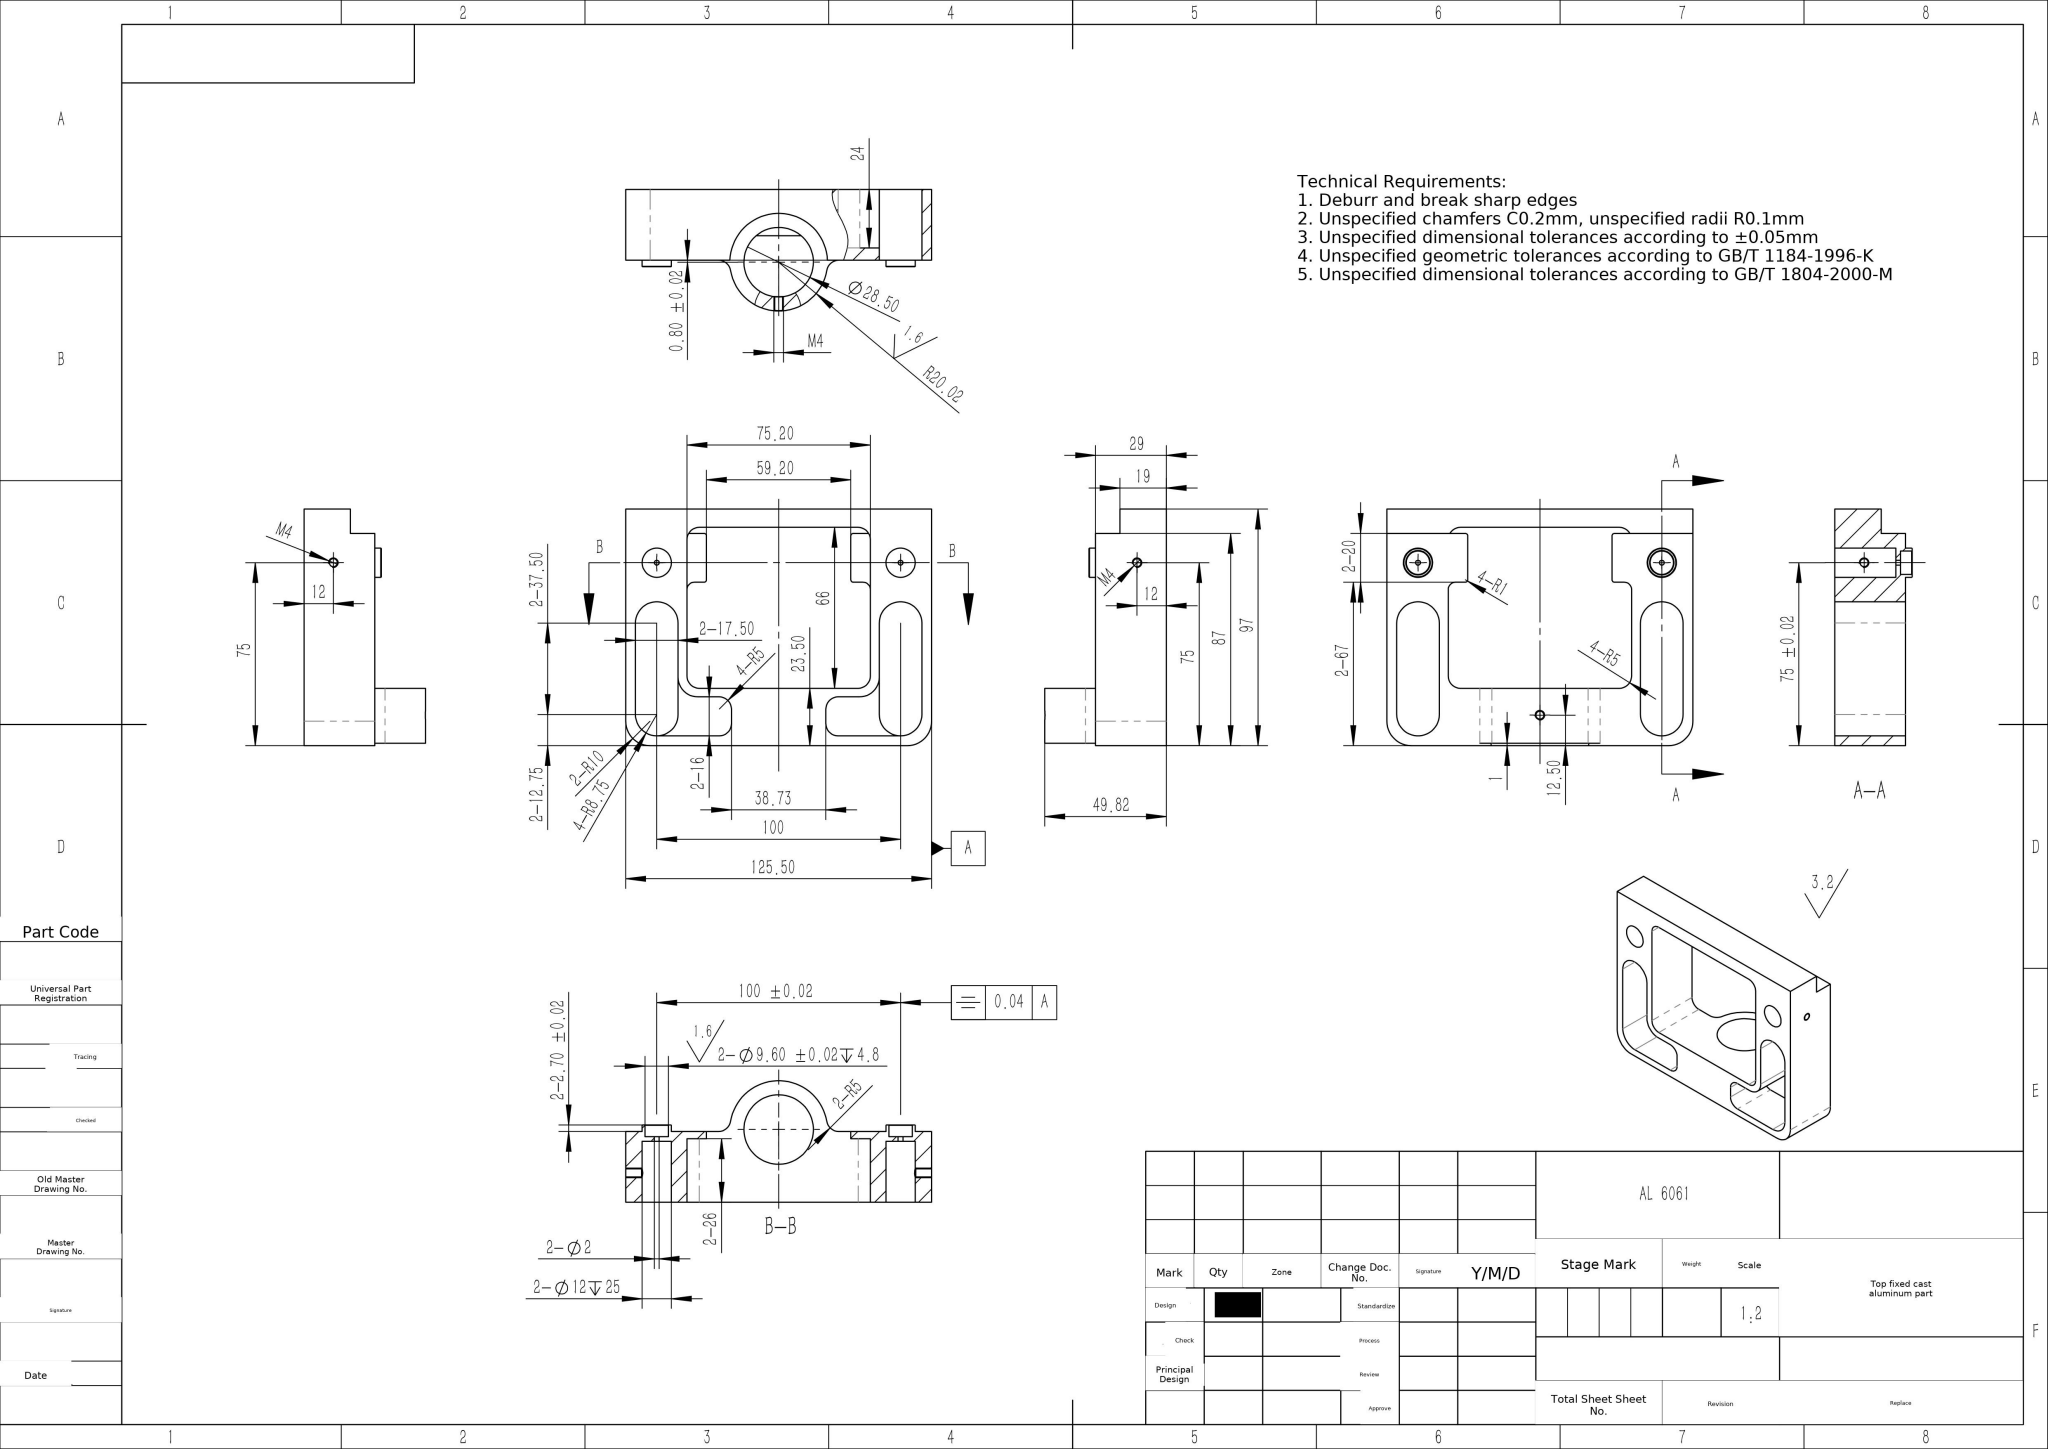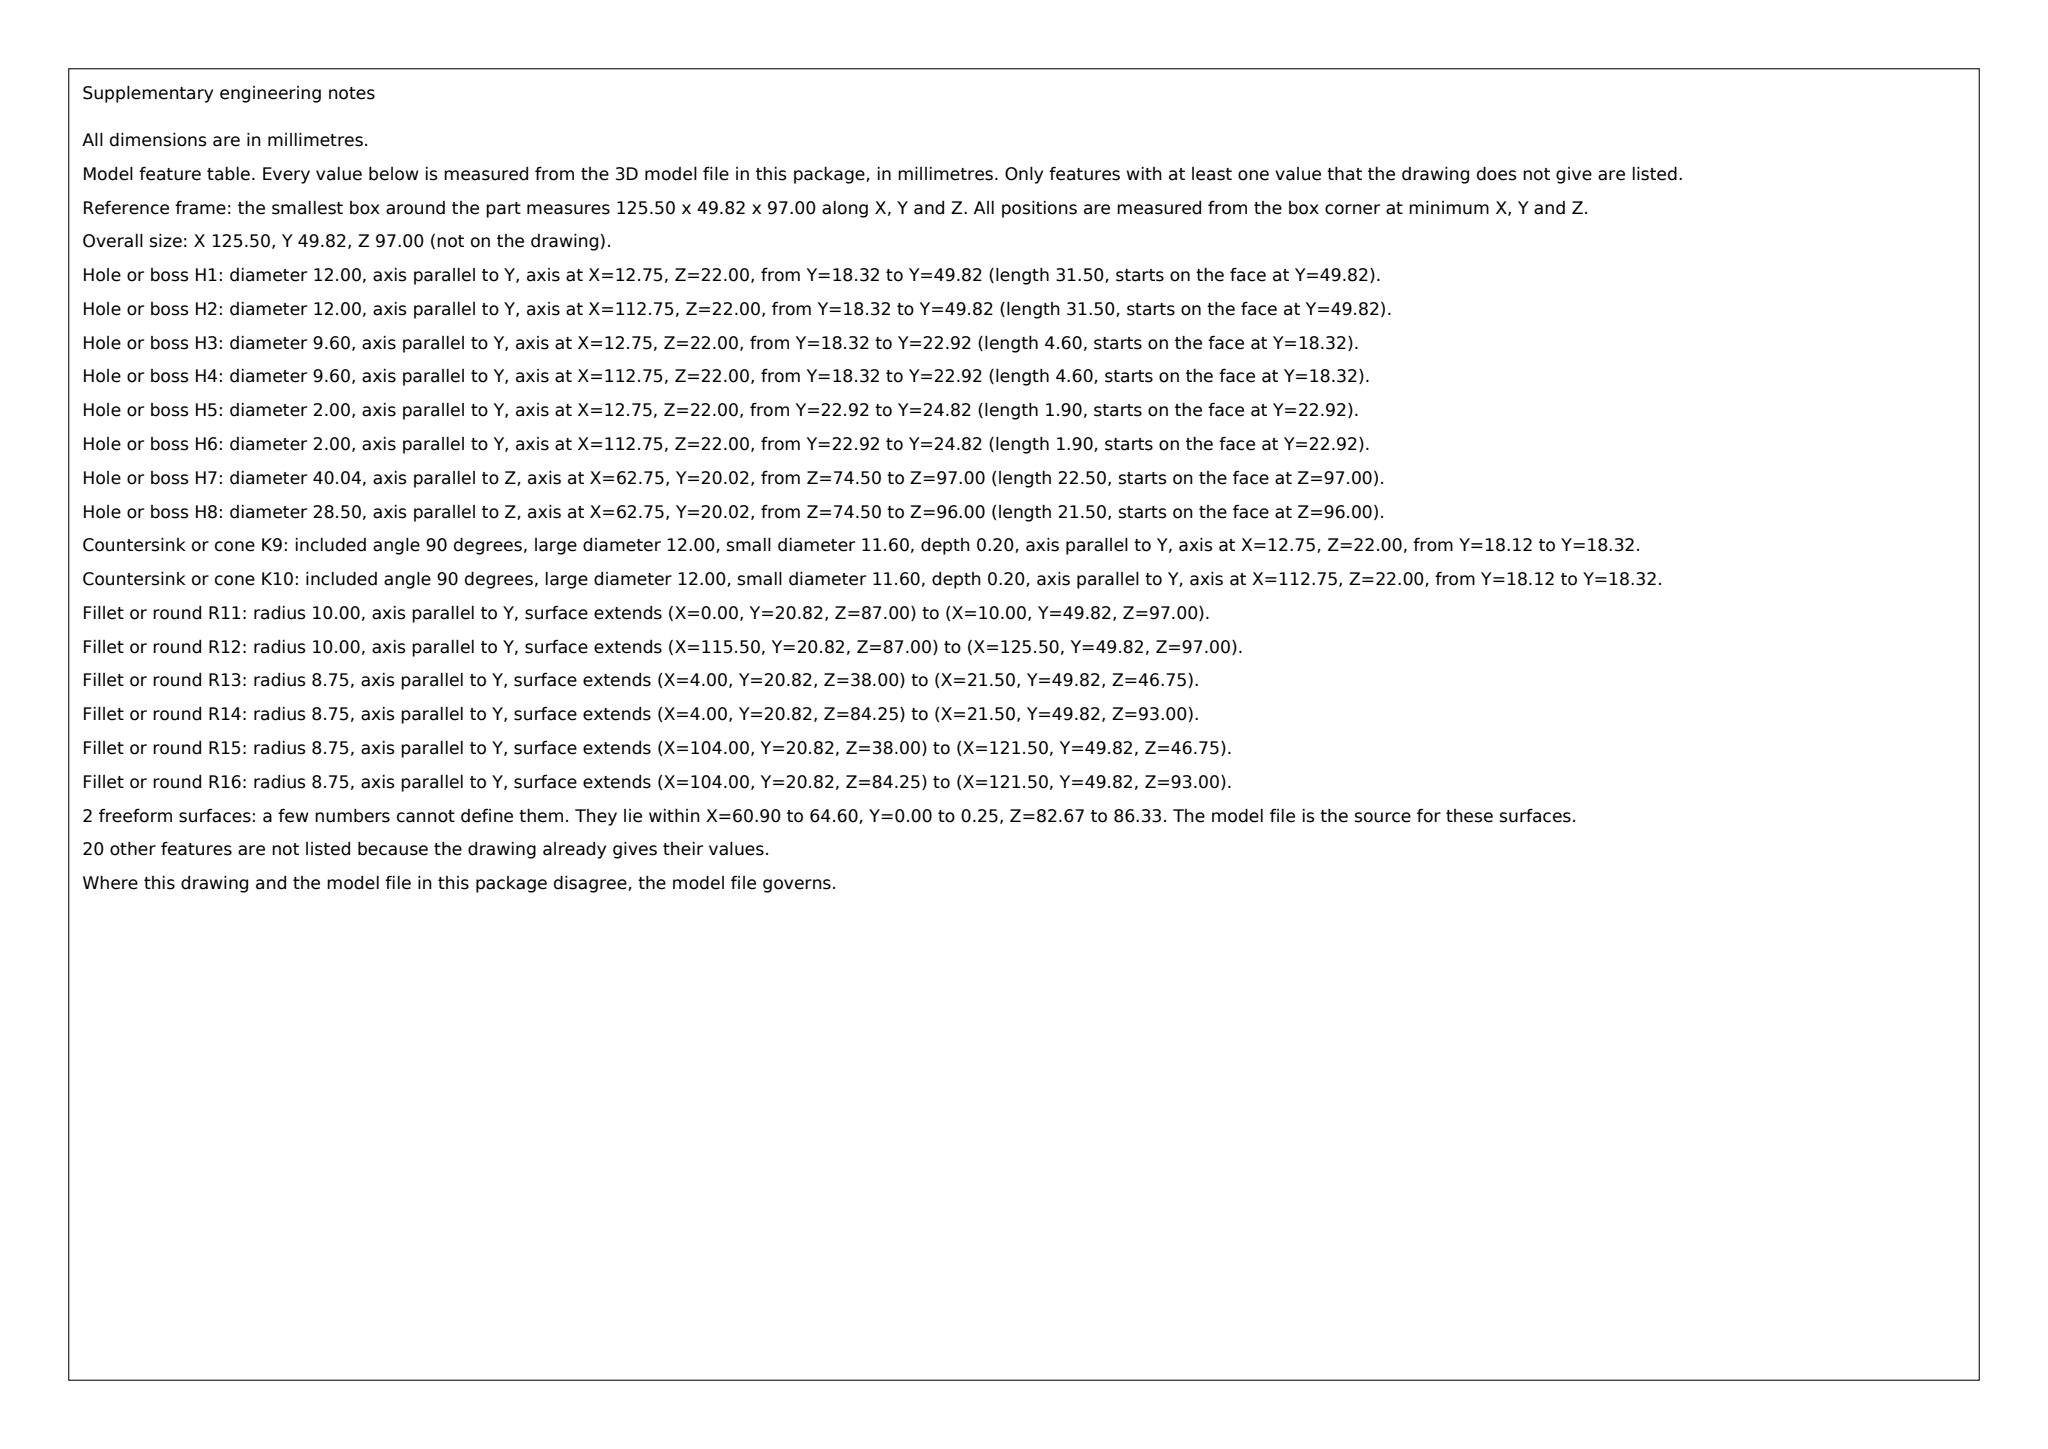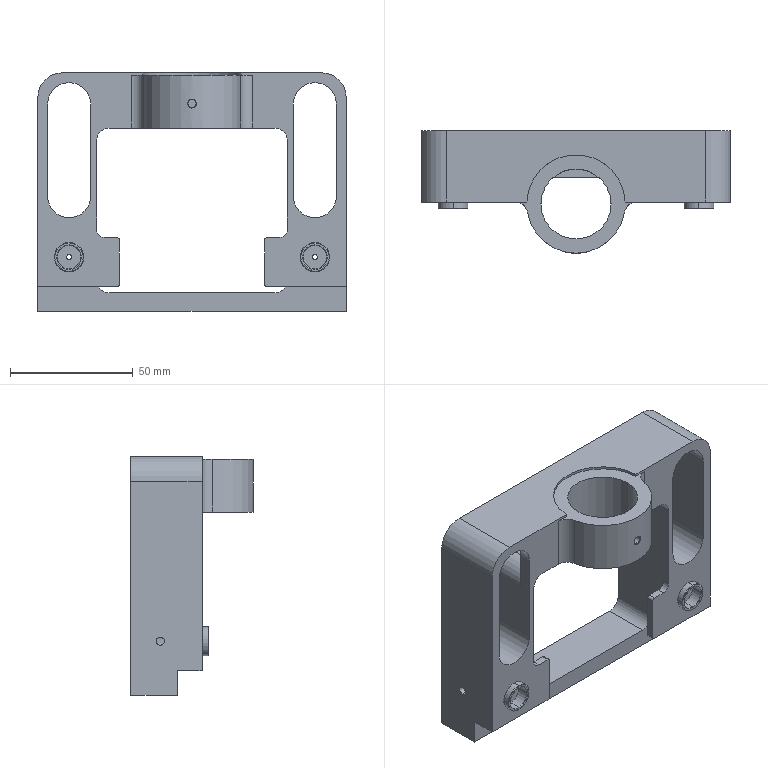Part | SolidWorks | mm | material AL 6061 | 1 solid | 101 faces | box 125.5 x 49.82 x 97 mm | volume 116626 mm3 | cylinder 52 | plane 39 | cone 8 | spline 2 | commonest cylinder face diameters 10 x10 12 x8 2 x8 3.3 x6 17.5 x6 9.6 x4 28.5 x2 20 x2